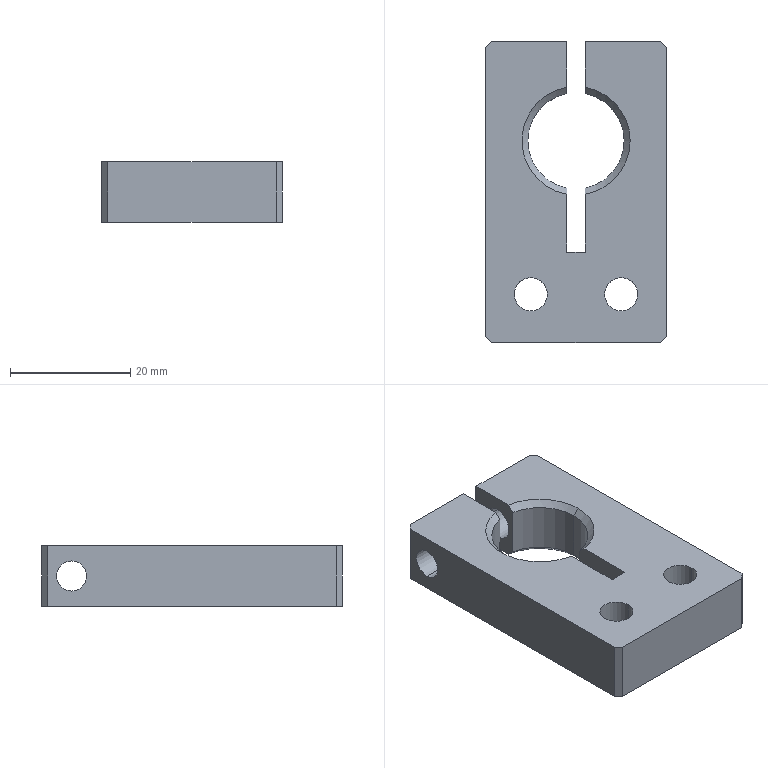Component | SolidWorks | SL010-LeftStreamline-1-1_SL010-2M-0112-000-2-1-1_SL010-LXFB-0102011-1-1 | 1 solid | 39 faces | box 30 x 50 x 10 mm | volume 10698 mm3 | plane 18 | cylinder 15 | cone 6 | commonest cylinder face diameters 5.5 x6 10 x4 16 x3 5 x2 | material Aluminum-6061
build123d program:
from build123d import *

# Parameters (mm, degrees)
SKETCH1_W                                       = 30
SKETCH1_H                                       = 50
BOSS_EXTRUDE1_DEPTH                             = 5
SKETCH2_R                                       = 8
CUT_EXTRUDE1_DEPTH                              = 31.822
CHAMFER2_SIZE                                   = 1
SKETCH3_W                                       = 3
SKETCH3_H                                       = 70
CUT_EXTRUDE2_DEPTH                              = 31.822
CUT_EXTRUDE3_REACH                              = 41.37
SKETCH4_R                                       = 2.75
M5_TAPPED_HOLE1_D                               = 5
M5_HEX_SOCKET_HEAD_CAP_SCREW_CBORE1_D           = 5.5
M5_HEX_SOCKET_HEAD_CAP_SCREW_CBORE1_CBORE_D     = 10
M5_HEX_SOCKET_HEAD_CAP_SCREW_CBORE1_CBORE_DEPTH = 5.4
CHAMFER1_SIZE                                   = 1


with BuildPart() as part:
    # Sketch1 → Boss-Extrude1 (new, symmetric)
    with BuildSketch(Plane.XY):
        Rectangle(SKETCH1_W, SKETCH1_H)
    extrude(amount=BOSS_EXTRUDE1_DEPTH, both=True)

    # Sketch2 → Cut-Extrude1 (cut, through all)
    with BuildSketch(Plane.XY.offset(5)):
        with Locations((0, 8.5)):
            Circle(SKETCH2_R)
    extrude(amount=-CUT_EXTRUDE1_DEPTH, mode=Mode.SUBTRACT)

    # Chamfer2
    chamfer2_edges = [part.edges().sort_by_distance(p)[0] for p in [
        (-8, 8.5, -5),
        (-8, 8.5, 5),
    ]]
    chamfer(chamfer2_edges, length=CHAMFER2_SIZE)

    # Sketch3 → Cut-Extrude2 (cut, through all)
    with BuildSketch(Plane.XY.offset(5)):
        with Locations((0, 25)):
            Rectangle(SKETCH3_W, SKETCH3_H)
    extrude(amount=-CUT_EXTRUDE2_DEPTH, mode=Mode.SUBTRACT)

    # Sketch4 → Cut-Extrude3 (cut, up to next)
    with BuildSketch(Plane(origin=(15, 0, 0), x_dir=(0, 0, -1), z_dir=(1, 0, 0)), mode=Mode.PRIVATE) as cut_extrude3_sk1:
        with Locations(Location((0, 20, 0), (0, 0, 90))):
            Circle(SKETCH4_R)
    cut_extrude3_tool1 = extrude(cut_extrude3_sk1.sketch, amount=-CUT_EXTRUDE3_REACH, mode=Mode.PRIVATE) & part.part
    add(cut_extrude3_tool1.solids().sort_by_distance((15, 20, 0))[0], mode=Mode.SUBTRACT)

    # M5 Tapped Hole1 (through all)
    with Locations(Plane(origin=(-1.5, 0, 0), x_dir=(0, 0, -1), z_dir=(1, 0, 0))):
        with Locations((0, 20)):
            Hole(M5_TAPPED_HOLE1_D / 2)

    # M5 Hex Socket Head Cap Screw CBORE1 (through all)
    with Locations(Plane(origin=(-9.711, 1.225, -5), x_dir=(1, 0, 0), z_dir=(0, 0, -1))):
        with Locations((2.211, 18.225), (17.211, 18.225)):
            CounterBoreHole(M5_HEX_SOCKET_HEAD_CAP_SCREW_CBORE1_D / 2, M5_HEX_SOCKET_HEAD_CAP_SCREW_CBORE1_CBORE_D / 2, M5_HEX_SOCKET_HEAD_CAP_SCREW_CBORE1_CBORE_DEPTH)

    # Chamfer1
    chamfer1_edges = [part.edges().sort_by_distance(p)[0] for p in [
        (15, -25, 0),
        (-15, -25, 0),
        (-15, 25, 0),
        (15, 25, 0),
    ]]
    chamfer(chamfer1_edges, length=CHAMFER1_SIZE)


solid = part.part

# Placed as in the assembly
solid = solid.moved(Location((-175, -173.404, -718.035), (0, 0, 0)))